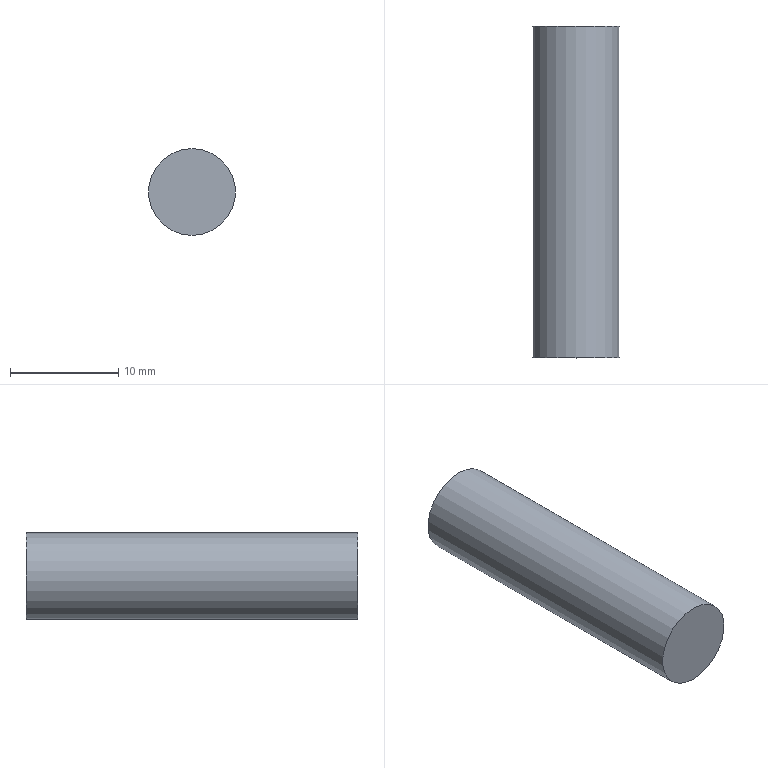Component | NX | CONN_PIN | 1 solid | 3 faces | box 8 x 30.6 x 8 mm | volume 1538 mm3 | plane 2 | cylinder 1 | commonest cylinder face diameters 8 x1
STEP:
#1=CARTESIAN_POINT('',(0.,0.,0.));
#2=DIRECTION('',(0.,0.,1.));
#3=DIRECTION('',(1.,0.,0.));
#4=AXIS2_PLACEMENT_3D('',#1,#2,#3);
#5=CARTESIAN_POINT('',(-71.853,-7.5,216.59));
#6=VERTEX_POINT('',#5);
#7=CARTESIAN_POINT('',(-71.853,-7.5,220.59));
#8=DIRECTION('',(0.,1.,0.));
#9=DIRECTION('',(0.,0.,-1.));
#10=AXIS2_PLACEMENT_3D('',#7,#8,#9);
#11=CIRCLE('',#10,4.);
#12=CARTESIAN_POINT('',(-71.853,-10.,220.59));
#13=DIRECTION('',(0.,1.,0.));
#14=DIRECTION('',(0.,0.,1.));
#15=AXIS2_PLACEMENT_3D('',#12,#13,#14);
#16=CYLINDRICAL_SURFACE('',#15,4.);
#17=CARTESIAN_POINT('',(3.142,2.5));
#18=DIRECTION('',(1.,0.));
#19=VECTOR('',#18,1.);
#20=LINE('',#17,#19);
#21=(GEOMETRIC_REPRESENTATION_CONTEXT(2)PARAMETRIC_REPRESENTATION_CONTEXT()REPRESENTATION_CONTEXT('',''));
#22=DEFINITIONAL_REPRESENTATION('',(#20),#21);
#23=PCURVE('',#16,#22);
#24=CARTESIAN_POINT('',(-71.853,-7.5,220.59));
#25=DIRECTION('',(0.,1.,0.));
#26=DIRECTION('',(0.,0.,1.));
#27=AXIS2_PLACEMENT_3D('',#24,#25,#26);
#28=PLANE('',#27);
#29=CARTESIAN_POINT('',(0.,0.));
#30=DIRECTION('',(-1.,0.));
#31=AXIS2_PLACEMENT_2D('',#29,#30);
#32=CIRCLE('',#31,4.);
#33=(GEOMETRIC_REPRESENTATION_CONTEXT(2)PARAMETRIC_REPRESENTATION_CONTEXT()REPRESENTATION_CONTEXT('',''));
#34=DEFINITIONAL_REPRESENTATION('',(#32),#33);
#35=PCURVE('',#28,#34);
#36=SURFACE_CURVE('',#11,(#23,#35),.PCURVE_S1.);
#37=EDGE_CURVE('',#6,#6,#36,.T.);
#38=ORIENTED_EDGE('',*,*,#37,.T.);
#39=CARTESIAN_POINT('',(-71.853,23.1,216.59));
#40=VERTEX_POINT('',#39);
#41=CARTESIAN_POINT('',(-71.853,-7.5,216.59));
#42=CARTESIAN_POINT('',(-71.853,23.1,216.59));
#43=B_SPLINE_CURVE_WITH_KNOTS('',1,(#41,#42),.UNSPECIFIED.,.F.,.F.,(2,2),(2.5,33.1),.PIECEWISE_BEZIER_KNOTS.);
#44=CARTESIAN_POINT('',(9.425,0.));
#45=DIRECTION('',(0.,1.));
#46=VECTOR('',#45,1.);
#47=LINE('',#44,#46);
#48=(GEOMETRIC_REPRESENTATION_CONTEXT(2)PARAMETRIC_REPRESENTATION_CONTEXT()REPRESENTATION_CONTEXT('',''));
#49=DEFINITIONAL_REPRESENTATION('',(#47),#48);
#50=PCURVE('',#16,#49);
#51=CARTESIAN_POINT('',(3.142,0.));
#52=DIRECTION('',(0.,1.));
#53=VECTOR('',#52,1.);
#54=LINE('',#51,#53);
#55=(GEOMETRIC_REPRESENTATION_CONTEXT(2)PARAMETRIC_REPRESENTATION_CONTEXT()REPRESENTATION_CONTEXT('',''));
#56=DEFINITIONAL_REPRESENTATION('',(#54),#55);
#57=PCURVE('',#16,#56);
#58=SEAM_CURVE('',#43,(#50,#57),.PCURVE_S1.);
#59=EDGE_CURVE('',#6,#40,#58,.T.);
#60=ORIENTED_EDGE('',*,*,#59,.T.);
#61=CARTESIAN_POINT('',(-71.853,23.1,220.59));
#62=DIRECTION('',(0.,1.,0.));
#63=DIRECTION('',(0.,0.,-1.));
#64=AXIS2_PLACEMENT_3D('',#61,#62,#63);
#65=CIRCLE('',#64,4.);
#66=CARTESIAN_POINT('',(3.142,33.1));
#67=DIRECTION('',(1.,0.));
#68=VECTOR('',#67,1.);
#69=LINE('',#66,#68);
#70=(GEOMETRIC_REPRESENTATION_CONTEXT(2)PARAMETRIC_REPRESENTATION_CONTEXT()REPRESENTATION_CONTEXT('',''));
#71=DEFINITIONAL_REPRESENTATION('',(#69),#70);
#72=PCURVE('',#16,#71);
#73=CARTESIAN_POINT('',(-71.853,23.1,220.59));
#74=DIRECTION('',(0.,1.,0.));
#75=DIRECTION('',(0.,0.,1.));
#76=AXIS2_PLACEMENT_3D('',#73,#74,#75);
#77=PLANE('',#76);
#78=CARTESIAN_POINT('',(0.,0.));
#79=DIRECTION('',(-1.,0.));
#80=AXIS2_PLACEMENT_2D('',#78,#79);
#81=CIRCLE('',#80,4.);
#82=(GEOMETRIC_REPRESENTATION_CONTEXT(2)PARAMETRIC_REPRESENTATION_CONTEXT()REPRESENTATION_CONTEXT('',''));
#83=DEFINITIONAL_REPRESENTATION('',(#81),#82);
#84=PCURVE('',#77,#83);
#85=SURFACE_CURVE('',#65,(#72,#84),.PCURVE_S1.);
#86=EDGE_CURVE('',#40,#40,#85,.T.);
#87=ORIENTED_EDGE('',*,*,#86,.F.);
#88=ORIENTED_EDGE('',*,*,#59,.F.);
#89=EDGE_LOOP('',(#38,#60,#87,#88));
#90=FACE_BOUND('',#89,.T.);
#91=ADVANCED_FACE('',(#90),#16,.T.);
#92=ORIENTED_EDGE('',*,*,#37,.F.);
#93=EDGE_LOOP('',(#92));
#94=FACE_BOUND('',#93,.T.);
#95=ADVANCED_FACE('',(#94),#28,.F.);
#96=ORIENTED_EDGE('',*,*,#86,.T.);
#97=EDGE_LOOP('',(#96));
#98=FACE_BOUND('',#97,.T.);
#99=ADVANCED_FACE('',(#98),#77,.T.);
#100=CLOSED_SHELL('',(#91,#95,#99));
#101=MANIFOLD_SOLID_BREP('',#100);
#102=(LENGTH_UNIT()NAMED_UNIT(*)SI_UNIT(.MILLI.,.METRE.));
#103=UNCERTAINTY_MEASURE_WITH_UNIT(LENGTH_MEASURE(0.00001),#102,'','');
#104=(NAMED_UNIT(*)PLANE_ANGLE_UNIT()SI_UNIT($,.RADIAN.));
#105=(NAMED_UNIT(*)SI_UNIT($,.STERADIAN.)SOLID_ANGLE_UNIT());
#106=(GEOMETRIC_REPRESENTATION_CONTEXT(3)GLOBAL_UNCERTAINTY_ASSIGNED_CONTEXT((#103))GLOBAL_UNIT_ASSIGNED_CONTEXT((#102,#104,#105))REPRESENTATION_CONTEXT('',''));
#107=ADVANCED_BREP_SHAPE_REPRESENTATION('',(#4,#101),#106);